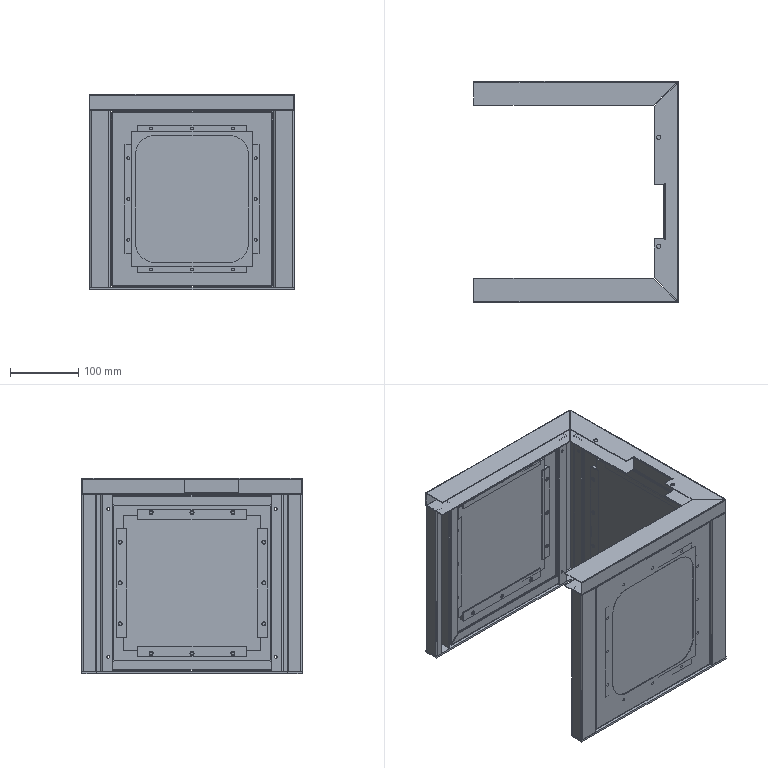Assembly | SolidWorks | mm | 36 component files | 36 solids | 832 faces | box 300 x 324 x 286.4 mm | volume 1127977 mm3 | plane 486 | cylinder 290 | spline 56 | commonest cylinder face diameters 4.2 x88 6 x84 0.1 x49 2.5 x33 4.1 x16 60 x12 10 x8
Bill of materials:
Cover1-2XG1 | 2 |  | Long, straight, constant-wall bent profile. The cross-section has a rectangular box-like centre with rounded corners and two offset flanges that run out in perpendicular directions. One flange has two small through-holes, one near each end.
Cover1-3XG1 | 2 |  | Flat square plate with one large central rectangular cutout with rounded corners, which leaves a frame of fairly even width.
Cover1-4XG1 | 1 |  | Flat rectangular plate frame with a large central opening with rounded corners and four small through-holes, one near each outer corner.
Cover1-5-2XG1 | 1 |  | Plain thin rectangular flat plate with no holes or cutouts.
Cover1-5XG1 | 2 |  | Plain thin rectangular flat plate with no holes, close to square and slightly taller than wide.
Cover1-6XG1 | 12 |  | Long, narrow, rectangular bar with three evenly spaced round through-holes along the centreline of one face.
Cover1-7XG1 | 12 |  | Long, thin, flat strip with three evenly spaced round through-holes on one longitudinal line.
Cover1-8XG1 | 1 |  | Thick, flat, U-shaped frame plate: three straight arms with mitered corners, open on one side. One inner edge has a rectangular step notch, and there are two small holes near that notch.
Cover1-9XG1 | 1 |  | Thin, flat, U-shaped frame strip with square inside and outside corners, open on one side, with no holes.
Cover1XG1 | 2 |  | Long, straight, open channel profile with constant wall thickness and rounded outer corners. The section is a rounded rectangle left open along one side, with a short inward return lip on one leg only.
Mates:
1. coincident | Cover1XG1-1 face at (-150, 162, 260) dir (-1, 0, 0) | assembly sketch segment at (-150, 162, 0) dir (0, -1, 0)
2. coincident | Cover1XG1-1 face at (-150, 162, 260) dir (0, 1, 0) | assembly sketch segment at (-150, 162, 0) dir (1, 0, 0)
3. coincident | Cover1XG1-1 face at (-122, 159.95, 0) dir (0, 0, -1) | assembly plane at (0, 0, 0) dir (0, 0, 1)
4. coincident | Cover1-2XG1-1 face at (150, 162, 260) dir (1, 0, 0) | assembly sketch segment at (150, 162, 0) dir (0, -1, 0)
5. coincident | Cover1-2XG1-1 face at (150, 162, 260) dir (0, 1, 0) | assembly sketch segment at (-150, 162, 0) dir (1, 0, 0)
6. coincident | Cover1-2XG1-1 face at (148, 159.95, 0) dir (0, 0, -1) | assembly plane at (0, 0, 0) dir (0, 0, 1)
7. coincident | Cover1-3XG1-1 plane at (0, -158.8, 130) dir (1, 0, 0) | assembly plane at (0, 0, 0) dir (1, 0, 0)
8. distance | Cover1-3XG1-1 face at (0, -158.8, 1.5) dir (0, 0, -1) | assembly plane at (0, 0, 0) dir (0, 0, 1)
9. coincident | Cover1-2XG1-2 face at (120, -142, 0) dir (0, -1, 0) | Cover1-3XG1-1 face at (0, -142, 130) dir (0, 1, 0)
10. coincident | Cover1-4XG1-1 plane at (146.8, 0, 130) dir (0, 1, 0) | assembly plane at (0, 0, 0) dir (0, 1, 0)
11. distance | Cover1-4XG1-1 face at (146.8, 0, 1.5) dir (0, 0, -1) | assembly plane at (0, 0, 0) dir (0, 0, 1)
12. coincident | Cover1-2XG1-1 face at (130, 132, 260) dir (1, 0, 0) | Cover1-4XG1-1 face at (130, 0, 130) dir (-1, 0, 0)
13. coincident | Cover1-3XG1-1 plane at (0, -158.8, 130) dir (0, 0, 1) | Cover1-5XG1-1 plane at (0, -158.8, 130) dir (0, 0, -1)
14. coincident | Cover1-3XG1-1 plane at (0, -158.8, 130) dir (1, 0, 0) | Cover1-5XG1-1 plane at (0, -158.8, 130) dir (1, 0, 0)
15. coincident | Cover1-3XG1-1 face at (0, -158.8, 130) dir (0, 1, 0) | Cover1-5XG1-1 face at (0, -158.8, 130) dir (0, -1, 0)
16. coincident | Cover1-3XG1-1 plane at (0, -158.8, 130) dir (0, 0, 1) | Cover1-6XG1-1 plane at (93.5, -154.8, 130) dir (0, 0, -1)
17. coincident | Cover1-3XG1-1 face at (0, -158.8, 130) dir (0, 1, 0) | Cover1-6XG1-1 face at (93.5, -158.8, 130) dir (0, -1, 0)
18. coincident | Cover1-5XG1-1 face at (88.5, -154.8, 31.5) dir (1, 0, 0) | Cover1-6XG1-1 face at (88.5, -158.8, 210) dir (-1, 0, 0)
19. coincident | Cover1-3XG1-1 plane at (0, -158.8, 130) dir (1, 0, 0) | Cover1-6XG1-2 plane at (0, -154.8, 233.5) dir (1, 0, 0)
20. coincident | Cover1-3XG1-1 face at (0, -158.8, 130) dir (0, 1, 0) | Cover1-6XG1-2 face at (0, -158.8, 233.5) dir (0, -1, 0)
21. coincident | Cover1-5XG1-1 face at (-88.5, -154.8, 228.5) dir (0, 0, 1) | Cover1-6XG1-2 face at (-80, -158.8, 228.5) dir (0, 0, -1)
22. concentric | Cover1-6XG1-4 face at (60, -154.8, 26.5) dir (0, 1, 0) r 2.1 | Cover1-7XG1-1 face at (60, -153.3, 26.5) dir (0, -1, 0) r 3
23. concentric | Cover1-6XG1-4 face at (-60, -154.8, 26.5) dir (0, 1, 0) r 2.1 | Cover1-7XG1-1 face at (-60, -153.3, 26.5) dir (0, -1, 0) r 3
24. coincident | Cover1-6XG1-4 face at (0, -154.8, 26.5) dir (0, 1, 0) | Cover1-7XG1-1 face at (0, -154.8, 29) dir (0, -1, 0)
25. concentric | Cover1-6XG1-3 face at (-93.5, -154.8, 70) dir (0, 1, 0) r 2.1 | Cover1-7XG1-2 face at (-93.5, -153.3, 70) dir (0, -1, 0) r 3
26. concentric | Cover1-6XG1-3 face at (-93.5, -154.8, 190) dir (0, 1, 0) r 2.1 | Cover1-7XG1-2 face at (-93.5, -153.3, 190) dir (0, -1, 0) r 3
27. coincident | Cover1-6XG1-3 face at (-93.5, -154.8, 130) dir (0, 1, 0) | Cover1-7XG1-2 face at (-91, -154.8, 130) dir (0, -1, 0)
28. concentric | Cover1-6XG1-2 face at (-60, -158.8, 233.5) dir (0, -1, 0) r 2.1 | Cover1-7XG1-4 face at (-60, -153.3, 233.5) dir (0, -1, 0) r 3
29. concentric | Cover1-6XG1-2 face at (60, -158.8, 233.5) dir (0, -1, 0) r 2.1 | Cover1-7XG1-4 face at (60, -153.3, 233.5) dir (0, -1, 0) r 3
30. coincident | Cover1-6XG1-2 face at (0, -154.8, 233.5) dir (0, 1, 0) | Cover1-7XG1-4 face at (0, -154.8, 231) dir (0, -1, 0)
31. concentric | Cover1-6XG1-1 face at (93.5, -158.8, 190) dir (0, -1, 0) r 2.1 | Cover1-7XG1-6 face at (93.5, -153.3, 190) dir (0, -1, 0) r 3
32. concentric | Cover1-6XG1-1 face at (93.5, -158.8, 70) dir (0, -1, 0) r 2.1 | Cover1-7XG1-6 face at (93.5, -153.3, 70) dir (0, -1, 0) r 3
33. coincident | Cover1-6XG1-1 face at (93.5, -154.8, 130) dir (0, 1, 0) | Cover1-7XG1-6 face at (91, -154.8, 130) dir (0, -1, 0)
34. coincident | Cover1-8XG1-1 plane at (150, 0, 271.7) dir (0, 1, 0) | assembly plane at (0, 0, 0) dir (0, 1, 0)
35. coincident | Cover1-2XG1-1 face at (150, 162, 260) dir (1, 0, 0) | Cover1-8XG1-1 face at (150, -162, 282.2) dir (1, 0, 0)
36. coincident | Cover1-2XG1-1 face at (147.95, 160, 260) dir (0, 0, 1) | Cover1-8XG1-1 face at (150, 0, 260) dir (0, 0, -1)
37. coincident | Cover1-4XG1-1 plane at (146.8, 0, 130) dir (0, 1, 0) | Cover1-5-2XG1-1 plane at (146.8, 0, 130) dir (0, -1, 0)
38. coincident | Cover1-4XG1-1 plane at (146.8, 0, 130) dir (0, 0, 1) | Cover1-5-2XG1-1 plane at (146.8, 0, 130) dir (0, 0, 1)
39. coincident | Cover1-4XG1-1 face at (146.8, 0, 130) dir (-1, 0, 0) | Cover1-5-2XG1-1 face at (146.8, 0, 130) dir (1, 0, 0)
40. coincident | Cover1-6XG1-9 plane at (146.8, 0, 233.5) dir (0, -1, 0) | assembly plane at (0, 0, 0) dir (0, 1, 0)
41. coincident | Cover1-4XG1-1 face at (146.8, 0, 130) dir (-1, 0, 0) | Cover1-6XG1-9 face at (146.8, 0, 233.5) dir (1, 0, 0)
42. coincident | Cover1-5-2XG1-1 face at (142.8, 100.5, 228.5) dir (0, 0, 1) | Cover1-6XG1-9 face at (142.8, 80, 228.5) dir (0, 0, -1)
43. coincident | Cover1-4XG1-1 plane at (146.8, 0, 130) dir (0, 0, 1) | Cover1-6XG1-10 plane at (146.8, 105.5, 130) dir (0, 0, 1)
44. coincident | Cover1-4XG1-1 face at (146.8, 0, 130) dir (-1, 0, 0) | Cover1-6XG1-10 face at (146.8, 105.5, 130) dir (1, 0, 0)
45. coincident | Cover1-5-2XG1-1 face at (142.8, 100.5, 228.5) dir (0, 1, 0) | Cover1-6XG1-10 face at (142.8, 100.5, 50) dir (0, -1, 0)
46. concentric | Cover1-6XG1-9 face at (142.8, -60, 233.5) dir (-1, 0, 0) r 2.1 | Cover1-7XG1-11 face at (142.8, -60, 233.5) dir (-1, 0, 0) r 3
47. concentric | Cover1-6XG1-9 face at (142.8, 60, 233.5) dir (-1, 0, 0) r 2.1 | Cover1-7XG1-11 face at (142.8, 60, 233.5) dir (-1, 0, 0) r 3
48. coincident | Cover1-6XG1-9 face at (142.8, 0, 233.5) dir (-1, 0, 0) | Cover1-7XG1-11 face at (142.8, 0, 231) dir (1, 0, 0)
49. concentric | Cover1-6XG1-12 face at (146.8, -105.5, 70) dir (1, 0, 0) r 2.1 | Cover1-7XG1-12 face at (142.8, -105.5, 70) dir (-1, 0, 0) r 3
50. concentric | Cover1-6XG1-12 face at (146.8, -105.5, 190) dir (1, 0, 0) r 2.1 | Cover1-7XG1-12 face at (142.8, -105.5, 190) dir (-1, 0, 0) r 3
51. coincident | Cover1-6XG1-12 face at (142.8, -105.5, 130) dir (-1, 0, 0) | Cover1-7XG1-12 face at (142.8, -103, 130) dir (1, 0, 0)
52. concentric | Cover1-6XG1-11 face at (146.8, 60, 26.5) dir (1, 0, 0) r 2.1 | Cover1-7XG1-14 face at (142.8, 60, 26.5) dir (-1, 0, 0) r 3
53. concentric | Cover1-6XG1-11 face at (146.8, -60, 26.5) dir (1, 0, 0) r 2.1 | Cover1-7XG1-14 face at (142.8, -60, 26.5) dir (-1, 0, 0) r 3
54. coincident | Cover1-6XG1-11 face at (142.8, 0, 26.5) dir (-1, 0, 0) | Cover1-7XG1-14 face at (142.8, 0, 29) dir (1, 0, 0)
55. concentric | Cover1-6XG1-10 face at (142.8, 105.5, 190) dir (-1, 0, 0) r 2.1 | Cover1-7XG1-16 face at (142.8, 105.5, 190) dir (-1, 0, 0) r 3
56. concentric | Cover1-6XG1-10 face at (142.8, 105.5, 70) dir (-1, 0, 0) r 2.1 | Cover1-7XG1-16 face at (142.8, 105.5, 70) dir (-1, 0, 0) r 3
57. coincident | Cover1-6XG1-10 face at (142.8, 105.5, 130) dir (-1, 0, 0) | Cover1-7XG1-16 face at (142.8, 103, 130) dir (1, 0, 0)
58. coincident | Cover1-9XG1-1 plane at (150, 0, -3) dir (0, 1, 0) | assembly plane at (0, 0, 0) dir (0, 1, 0)
59. coincident | Cover1-9XG1-1 face at (150, -162, 0) dir (1, 0, 0) | Cover1-2XG1-1 face at (150, 162, 260) dir (1, 0, 0)
60. coincident | Cover1-2XG1-1 face at (147.95, 134, 0) dir (0, 0, -1) | Cover1-9XG1-1 face at (150, 0, 0) dir (0, 0, 1)